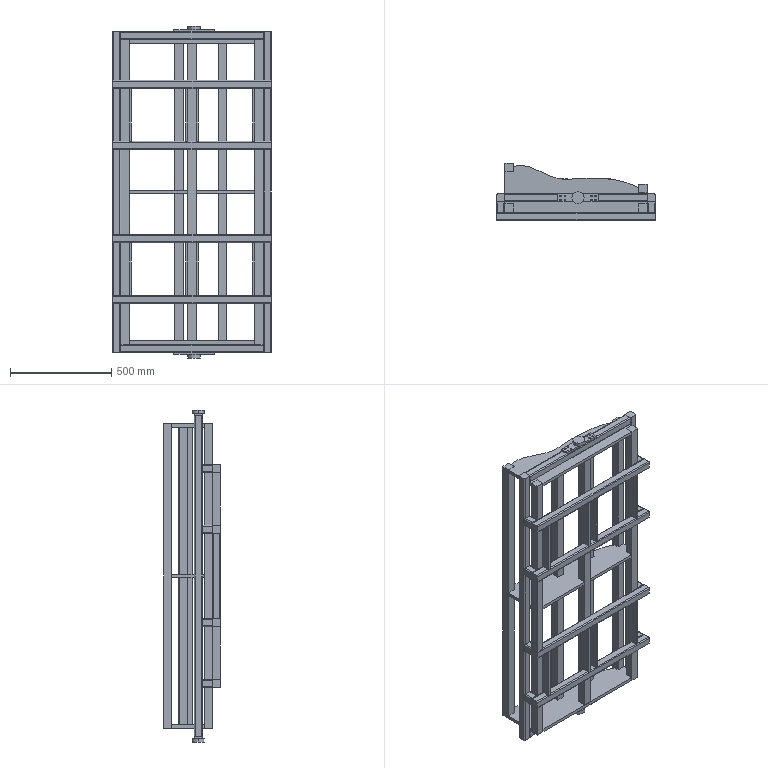Assembly | SolidWorks | mm | 37 component files | 37 solids | 434 faces | box 780 x 280 x 1636 mm | volume 37094171 mm3 | plane 293 | cylinder 104 | cone 32 | spline 5 | commonest cylinder face diameters 10 x68 6.147 x32 60 x4
Bill of materials:
Jig4040-1580 | 2 | Copper | Long, slender straight bar with a square cross-section and rounded longitudinal edges.
Jig4040-420 | 1 | Copper | Straight bar with a square cross-section and rounded longitudinal edges. It is stockier than unnamed part.
Jig4040-50 | 8 | Copper | Short block with a square cross-section and rounded longitudinal edges.
Jig4040-700 | 2 | Copper | Long, straight bar with a square cross-section and rounded longitudinal edges.
Jig4040-780 | 4 | Copper | Long, straight bar with a square cross-section and rounded longitudinal edges.
JigBaffle | 8 | Copper | Flat rectangular strip with both corners chamfered at one end, giving a tapered tip.
MiddlePlate | 1 |  | Thin flat plate with an irregular outline: curved, wavy edges, stepped rectangular tabs at both ends, and several rectangular notches along both long edges.
SidePlate | 2 |  | Thin flat plate with an irregular outline: a smooth wavy upper edge and stepped rectangular tabs at both ends. Unlike unnamed part, it has no notches between the ends.
SupportBar | 3 |  | Long, slender straight bar with a square cross-section and sharp edges.
TieRod | 4 |  | Long, slender straight bar with a square cross-section and sharp edges.
Two-AxisRotation | 2 |  | Flat rectangular plate with a raised cylindrical boss in the middle and eight small round holes, four at each end in a 2x2 pattern. The boss diameter is wider than the plate.
Mates:
1. coincident | Jig4040-1580-1 face at (11.992, -17.909, 2370) dir (1, 0, 0) | Jig4040-700-1 face at (11.992, 17.091, 2365) dir (-1, 0, 0)
2. coincident | Jig4040-1580-1 face at (-28.008, 22.091, 2370) dir (0, 1, 0) | Jig4040-700-1 face at (711.992, 22.091, 2365) dir (0, 1, 0)
3. coincident | Jig4040-1580-1 face at (-28.008, -17.909, 2370) dir (0, 0, 1) | Jig4040-700-1 face at (711.992, -12.909, 2370) dir (0, 0, 1)
4. coincident | Jig4040-1580-1 face at (-28.008, 22.091, 2370) dir (0, 1, 0) | Jig4040-700-2 face at (711.992, 22.091, 825) dir (0, 1, 0)
5. coincident | Jig4040-1580-1 face at (11.992, -17.909, 2370) dir (1, 0, 0) | Jig4040-700-2 face at (11.992, 17.091, 825) dir (-1, 0, 0)
6. coincident | Jig4040-1580-1 face at (-28.008, -17.909, 790) dir (0, 0, -1) | Jig4040-700-2 face at (711.992, -12.909, 790) dir (0, 0, -1)
7. coincident | Jig4040-700-1 face at (711.992, 22.091, 2365) dir (0, 1, 0) | Jig4040-1580-2 face at (711.992, 22.091, 2370) dir (0, 1, 0)
8. coincident | Jig4040-700-1 face at (711.992, -12.909, 2370) dir (0, 0, 1) | Jig4040-1580-2 face at (711.992, -17.909, 2370) dir (0, 0, 1)
9. coincident | Jig4040-700-1 face at (711.992, 17.091, 2365) dir (1, 0, 0) | Jig4040-1580-2 face at (711.992, -17.909, 2370) dir (-1, 0, 0)
10. coincident | Jig4040-700-1 face at (711.992, -12.909, 2330) dir (0, 0, -1) | SofaBackrest-1/SidePlate-2 face at (358.165, 95.613, 2330) dir (0, 0, 1)
11. coincident | Jig4040-1580-2 face at (711.992, -17.909, 2370) dir (-1, 0, 0) | SofaBackrest-1/TieRod-4 face at (711.992, 69.219, 2330) dir (1, 0, 0)
12. distance | SofaBackrest-1/TieRod-3 face at (671.992, -67.909, 2330) dir (0, -1, 0) | Jig4040-1580-2 face at (711.992, -17.909, 2370) dir (0, -1, 0)
13. coincident | Jig4040-1580-1 face at (-28.008, -17.909, 2370) dir (0, -1, 0) | Jig4040-50-1 face at (-23.008, -17.909, 2125) dir (0, 1, 0)
14. coincident | Jig4040-1580-1 face at (-28.008, -17.909, 2370) dir (-1, 0, 0) | Jig4040-50-1 face at (-28.008, -17.909, 2125) dir (-1, 0, 0)
15. coincident | Jig4040-1580-1 face at (-28.008, -17.909, 2370) dir (0, -1, 0) | Jig4040-50-2 face at (-23.008, -17.909, 1065) dir (0, 1, 0)
16. coincident | Jig4040-1580-1 face at (-28.008, -17.909, 2370) dir (-1, 0, 0) | Jig4040-50-2 face at (-28.008, -17.909, 1065) dir (-1, 0, 0)
17. distance | Jig4040-50-2 face at (-23.008, -17.909, 1030) dir (0, 0, -1) | Jig4040-1580-1 face at (-28.008, -17.909, 790) dir (0, 0, -1)
18. distance | Jig4040-50-1 face at (-23.008, -17.909, 2130) dir (0, 0, 1) | Jig4040-1580-1 face at (-28.008, -17.909, 2370) dir (0, 0, 1)
19. coincident | Jig4040-1580-1 face at (-28.008, -17.909, 2370) dir (0, -1, 0) | Jig4040-50-3 face at (-23.008, -17.909, 1365) dir (0, 1, 0)
20. coincident | Jig4040-50-2 face at (-28.008, -17.909, 1065) dir (-1, 0, 0) | Jig4040-50-3 face at (-28.008, -17.909, 1365) dir (-1, 0, 0)
21. coincident | Jig4040-1580-1 face at (-28.008, -17.909, 2370) dir (0, -1, 0) | Jig4040-50-4 face at (-23.008, -17.909, 1825) dir (0, 1, 0)
22. coincident | Jig4040-50-1 face at (-28.008, -17.909, 2125) dir (-1, 0, 0) | Jig4040-50-4 face at (-28.008, -17.909, 1825) dir (-1, 0, 0)
23. distance | Jig4040-50-4 face at (-23.008, -17.909, 1830) dir (0, 0, 1) | Jig4040-50-1 face at (-23.008, -17.909, 2090) dir (0, 0, -1)
24. distance | Jig4040-50-2 face at (-23.008, -17.909, 1070) dir (0, 0, 1) | Jig4040-50-3 face at (-23.008, -17.909, 1330) dir (0, 0, -1)
25. coincident | Jig4040-1580-2 face at (751.992, -17.909, 2370) dir (1, 0, 0) | Jig4040-50-5 face at (751.992, -17.909, 2125) dir (1, 0, 0)
26. coincident | Jig4040-1580-2 face at (711.992, -17.909, 2370) dir (0, -1, 0) | Jig4040-50-5 face at (716.992, -17.909, 2125) dir (0, 1, 0)
27. coincident | Jig4040-50-1 face at (-23.008, -17.909, 2130) dir (0, 0, 1) | Jig4040-50-5 face at (716.992, -17.909, 2130) dir (0, 0, 1)
28. coincident | Jig4040-1580-2 face at (751.992, -17.909, 2370) dir (1, 0, 0) | Jig4040-50-6 face at (751.992, -17.909, 1825) dir (1, 0, 0)
29. coincident | Jig4040-1580-2 face at (751.992, -17.909, 2370) dir (1, 0, 0) | Jig4040-50-7 face at (751.992, -17.909, 1365) dir (1, 0, 0)
30. coincident | Jig4040-1580-2 face at (751.992, -17.909, 2370) dir (1, 0, 0) | Jig4040-50-8 face at (751.992, -17.909, 1065) dir (1, 0, 0)
31. coincident | Jig4040-1580-2 face at (711.992, -17.909, 2370) dir (0, -1, 0) | Jig4040-50-6 face at (716.992, -17.909, 1825) dir (0, 1, 0)
32. coincident | Jig4040-1580-2 face at (711.992, -17.909, 2370) dir (0, -1, 0) | Jig4040-50-7 face at (716.992, -17.909, 1365) dir (0, 1, 0)
33. coincident | Jig4040-1580-2 face at (711.992, -17.909, 2370) dir (0, -1, 0) | Jig4040-50-8 face at (716.992, -17.909, 1065) dir (0, 1, 0)
34. coincident | Jig4040-50-2 face at (-23.008, -17.909, 1070) dir (0, 0, 1) | Jig4040-50-8 face at (716.992, -17.909, 1070) dir (0, 0, 1)
35. coincident | Jig4040-50-3 face at (-23.008, -17.909, 1370) dir (0, 0, 1) | Jig4040-50-7 face at (716.992, -17.909, 1370) dir (0, 0, 1)
36. coincident | Jig4040-50-4 face at (-23.008, -17.909, 1830) dir (0, 0, 1) | Jig4040-50-6 face at (716.992, -17.909, 1830) dir (0, 0, 1)
37. coincident | Jig4040-50-8 face at (716.992, -67.909, 1065) dir (0, -1, 0) | Jig4040-780-1 face at (-28.008, -67.909, 1035) dir (0, 1, 0)
38. coincident | Jig4040-50-8 face at (751.992, -17.909, 1065) dir (1, 0, 0) | Jig4040-780-1 face at (751.992, -102.909, 1035) dir (1, 0, 0)
39. coincident | Jig4040-50-8 face at (716.992, -17.909, 1070) dir (0, 0, 1) | Jig4040-780-1 face at (-28.008, -102.909, 1070) dir (0, 0, 1)
40. coincident | Jig4040-50-3 face at (-23.008, -67.909, 1365) dir (0, -1, 0) | Jig4040-780-2 face at (751.992, -67.909, 1365) dir (0, 1, 0)
41. coincident | Jig4040-50-3 face at (-23.008, -17.909, 1370) dir (0, 0, 1) | Jig4040-780-2 face at (751.992, -102.909, 1370) dir (0, 0, 1)
42. coincident | Jig4040-50-7 face at (751.992, -17.909, 1365) dir (1, 0, 0) | Jig4040-780-2 face at (751.992, -102.909, 1365) dir (1, 0, 0)
43. coincident | Jig4040-50-6 face at (716.992, -67.909, 1825) dir (0, -1, 0) | Jig4040-780-3 face at (751.992, -67.909, 1825) dir (0, 1, 0)
44. coincident | Jig4040-50-4 face at (-23.008, -17.909, 1830) dir (0, 0, 1) | Jig4040-780-3 face at (751.992, -102.909, 1830) dir (0, 0, 1)
45. coincident | Jig4040-50-4 face at (-28.008, -17.909, 1825) dir (-1, 0, 0) | Jig4040-780-3 face at (-28.008, -102.909, 1825) dir (-1, 0, 0)
46. coincident | Jig4040-50-5 face at (716.992, -67.909, 2125) dir (0, -1, 0) | Jig4040-780-4 face at (751.992, -67.909, 2125) dir (0, 1, 0)
47. coincident | Jig4040-50-5 face at (716.992, -17.909, 2090) dir (0, 0, -1) | Jig4040-780-4 face at (751.992, -102.909, 2090) dir (0, 0, -1)
48. coincident | Jig4040-50-5 face at (751.992, -17.909, 2125) dir (1, 0, 0) | Jig4040-780-4 face at (751.992, -102.909, 2125) dir (1, 0, 0)
49. coincident | Jig4040-780-2 face at (751.992, -107.909, 1365) dir (0, -1, 0) | JigBaffle-1 face at (51.992, -107.909, 1330) dir (0, -1, 0)
50. coincident | Jig4040-780-2 face at (751.992, -102.909, 1330) dir (0, 0, -1) | JigBaffle-1 face at (51.992, -107.909, 1330) dir (0, 0, 1)
51. coincident | SofaBackrest-1/TieRod-2 face at (51.992, -27.909, 2330) dir (1, 0, 0) | JigBaffle-1 face at (51.992, -107.909, 1330) dir (-1, 0, 0)
52. coincident | Jig4040-780-1 face at (-28.008, -107.909, 1035) dir (0, -1, 0) | JigBaffle-2 face at (331.992, -107.909, 1330) dir (0, -1, 0)
53. coincident | Jig4040-780-2 face at (751.992, -102.909, 1330) dir (0, 0, -1) | JigBaffle-2 face at (331.992, -107.909, 1330) dir (0, 0, 1)
54. coincident | SofaBackrest-1/SupportBar-2 face at (341.992, -27.909, 2314) dir (-1, 0, 0) | JigBaffle-2 face at (341.992, -107.909, 1330) dir (1, 0, 0)
55. coincident | Jig4040-780-2 face at (751.992, -107.909, 1365) dir (0, -1, 0) | JigBaffle-3 face at (381.992, -107.909, 1330) dir (0, -1, 0)
56. coincident | Jig4040-780-1 face at (-28.008, -102.909, 1070) dir (0, 0, 1) | JigBaffle-3 face at (381.992, -107.909, 1070) dir (0, 0, -1)
57. coincident | SofaBackrest-1/SupportBar-2 face at (381.992, -27.909, 2314) dir (1, 0, 0) | JigBaffle-3 face at (381.992, -107.909, 1330) dir (-1, 0, 0)
58. coincident | Jig4040-780-1 face at (-28.008, -107.909, 1035) dir (0, -1, 0) | JigBaffle-4 face at (661.992, -107.909, 1330) dir (0, -1, 0)
59. coincident | Jig4040-780-1 face at (-28.008, -102.909, 1070) dir (0, 0, 1) | JigBaffle-4 face at (661.992, -107.909, 1070) dir (0, 0, -1)
60. coincident | SofaBackrest-1/TieRod-3 face at (671.992, -27.909, 2330) dir (-1, 0, 0) | JigBaffle-4 face at (671.992, -107.909, 1330) dir (1, 0, 0)
61. coincident | Jig4040-780-4 face at (751.992, -107.909, 2125) dir (0, -1, 0) | JigBaffle-5 face at (51.992, -107.909, 2090) dir (0, -1, 0)
62. coincident | Jig4040-780-3 face at (751.992, -102.909, 1830) dir (0, 0, 1) | JigBaffle-5 face at (51.992, -107.909, 1830) dir (0, 0, -1)
63. coincident | SofaBackrest-1/TieRod-2 face at (51.992, -27.909, 2330) dir (1, 0, 0) | JigBaffle-5 face at (51.992, -107.909, 2090) dir (-1, 0, 0)
64. coincident | Jig4040-700-1 face at (711.992, -12.909, 2370) dir (0, 0, 1) | Two-AxisRotation-1 face at (271.992, -17.909, 2370) dir (0, 0, -1)
65. coincident | Jig4040-700-1 face at (711.992, 22.091, 2365) dir (0, 1, 0) | Two-AxisRotation-1 face at (271.992, 22.091, 2380) dir (0, 1, 0)
66. distance | Two-AxisRotation-1 face at (271.992, -17.909, 2380) dir (-1, 0, 0) | Jig4040-1580-1 face at (-28.008, -17.909, 2370) dir (-1, 0, 0)
67. coincident | Jig4040-700-2 face at (711.992, -12.909, 790) dir (0, 0, -1) | Two-AxisRotation-2 face at (471.992, -17.909, 790) dir (0, 0, 1)
68. coincident | Jig4040-700-2 face at (711.992, 22.091, 825) dir (0, 1, 0) | Two-AxisRotation-2 face at (471.992, 22.091, 780) dir (0, 1, 0)
69. distance | Two-AxisRotation-2 face at (271.992, -17.909, 780) dir (-1, 0, 0) | Jig4040-1580-1 face at (-28.008, -17.909, 2370) dir (-1, 0, 0)
70. coincident | Jig4040-780-4 face at (751.992, -107.909, 2125) dir (0, -1, 0) | JigBaffle-6 face at (381.992, -107.909, 2090) dir (0, -1, 0)
71. coincident | Jig4040-780-4 face at (751.992, -102.909, 2090) dir (0, 0, -1) | JigBaffle-6 face at (381.992, -107.909, 2090) dir (0, 0, 1)
72. coincident | SofaBackrest-1/SupportBar-2 face at (381.992, -27.909, 2314) dir (1, 0, 0) | JigBaffle-6 face at (381.992, -107.909, 2090) dir (-1, 0, 0)
73. coincident | Jig4040-780-4 face at (751.992, -107.909, 2125) dir (0, -1, 0) | JigBaffle-7 face at (331.992, -107.909, 2090) dir (0, -1, 0)
74. coincident | Jig4040-780-3 face at (751.992, -102.909, 1830) dir (0, 0, 1) | JigBaffle-7 face at (331.992, -107.909, 1830) dir (0, 0, -1)
75. coincident | SofaBackrest-1/SupportBar-2 face at (341.992, -27.909, 2314) dir (-1, 0, 0) | JigBaffle-7 face at (341.992, -107.909, 2090) dir (1, 0, 0)
76. coincident | SofaBackrest-1/TieRod-3 face at (671.992, -27.909, 2330) dir (-1, 0, 0) | JigBaffle-8 face at (671.992, -107.909, 2090) dir (1, 0, 0)
77. coincident | Jig4040-780-3 face at (751.992, -102.909, 1830) dir (0, 0, 1) | JigBaffle-8 face at (661.992, -107.909, 1830) dir (0, 0, -1)
78. coincident | Jig4040-780-4 face at (751.992, -107.909, 2125) dir (0, -1, 0) | JigBaffle-8 face at (661.992, -107.909, 2090) dir (0, -1, 0)
79. coincident | Jig4040-780-2 face at (-28.008, -102.909, 1365) dir (-1, 0, 0) | Jig4040-420-1 face at (-28.008, -102.909, 1790) dir (-1, 0, 0)
80. coincident | Jig4040-780-3 face at (751.992, -102.909, 1790) dir (0, 0, -1) | Jig4040-420-1 face at (-23.008, -72.909, 1790) dir (0, 0, 1)
81. coincident | Jig4040-780-2 face at (751.992, -107.909, 1365) dir (0, -1, 0) | Jig4040-420-1 face at (-23.008, -107.909, 1790) dir (0, -1, 0)
82. coincident | SidePlate-1 face at (-71.948, 36.297, -8) dir (0, 0, -1) | TieRod-1 face at (-385.456, 94.081, -8) dir (0, 0, -1)
83. coincident | SidePlate-1 face at (-418.121, -87.225, 8) dir (-1, 0, 0) | TieRod-1 face at (-418.121, 112.775, 1492) dir (-1, 0, 0)
84. coincident | SidePlate-1 face at (-418.121, 72.775, 8) dir (0, 1, 0) | TieRod-1 face at (-418.121, 72.775, 1492) dir (0, -1, 0)
85. coincident | SidePlate-1 face at (-418.121, -87.225, 8) dir (0, -1, 0) | TieRod-2 face at (-418.121, -87.225, 1492) dir (0, 1, 0)
86. coincident | SidePlate-1 face at (-418.121, -87.225, 8) dir (-1, 0, 0) | TieRod-2 face at (-418.121, -87.225, 1492) dir (-1, 0, 0)
87. coincident | SidePlate-1 face at (-71.948, 36.297, -8) dir (0, 0, -1) | TieRod-2 face at (-385.456, -105.919, -8) dir (0, 0, -1)
88. coincident | SidePlate-1 face at (281.879, -30.097, 8) dir (1, 0, 0) | TieRod-4 face at (281.879, 9.903, 1492) dir (1, 0, 0)
89. coincident | SidePlate-1 face at (-71.948, 36.297, -8) dir (0, 0, -1) | TieRod-4 face at (274.544, -8.79, -8) dir (0, 0, -1)
90. coincident | SidePlate-1 face at (281.879, -30.097, 8) dir (1, 0, 0) | TieRod-3 face at (281.879, -87.225, 1492) dir (1, 0, 0)
91. coincident | SidePlate-1 face at (-71.948, 36.297, -8) dir (0, 0, -1) | TieRod-3 face at (274.544, -105.919, -8) dir (0, 0, -1)
92. coincident | SidePlate-1 face at (-378.121, -127.225, 8) dir (0, -1, 0) | TieRod-3 face at (241.879, -127.225, 1492) dir (0, -1, 0)
93. coincident | SidePlate-1 face at (281.879, -30.097, 8) dir (0, 1, 0) | TieRod-4 face at (241.879, -30.097, 1492) dir (0, -1, 0)
94. coincident | TieRod-1 face at (-385.456, 94.081, 1492) dir (0, 0, 1) | SidePlate-2 face at (-71.948, 36.297, 1492) dir (0, 0, 1)
95. coincident | TieRod-2 face at (-418.121, -127.225, 1492) dir (0, -1, 0) | SidePlate-2 face at (-378.121, -127.225, 1492) dir (0, -1, 0)
96. coincident | TieRod-2 face at (-418.121, -87.225, 1492) dir (-1, 0, 0) | SidePlate-2 face at (-418.121, -87.225, 1492) dir (-1, 0, 0)
97. coincident | TieRod-2 face at (-418.121, -87.225, 1492) dir (-1, 0, 0) | MiddlePlate-1 face at (-418.121, -87.225, 750) dir (-1, 0, 0)
98. coincident | TieRod-2 face at (-418.121, -127.225, 1492) dir (0, -1, 0) | MiddlePlate-1 face at (-378.121, -127.225, 750) dir (0, -1, 0)
99. distance | MiddlePlate-1 face at (-264.174, 82.239, 750) dir (0, 0, 1) | SidePlate-2 face at (-71.948, 36.297, 1476) dir (0, 0, -1)
100. coincident | SupportBar-1 face at (-119.629, 17.592, 1476) dir (0, 0, 1) | SupportBar-2 face at (-55.456, -105.919, 1476) dir (0, 0, 1)
101. coincident | SupportBar-2 face at (-55.456, -105.919, 1476) dir (0, 0, 1) | SupportBar-3 face at (94.51, 20.069, 1476) dir (0, 0, 1)
102. coincident | SidePlate-2 face at (-71.948, 36.297, 1476) dir (0, 0, -1) | SupportBar-2 face at (-55.456, -105.919, 1476) dir (0, 0, 1)
103. coincident | MiddlePlate-1 face at (-152.294, 36.782, 750) dir (1, 0, 0) | SupportBar-1 face at (-152.294, 36.286, 1476) dir (-1, 0, 0)
104. coincident | MiddlePlate-1 face at (-88.121, -127.225, 750) dir (1, 0, 0) | SupportBar-2 face at (-88.121, -87.225, 1476) dir (-1, 0, 0)
105. coincident | MiddlePlate-1 face at (61.845, 38.84, 750) dir (1, 0, 0) | SupportBar-3 face at (61.845, 38.763, 1476) dir (-1, 0, 0)
106. coincident | MiddlePlate-1 face at (-378.121, -127.225, 750) dir (0, -1, 0) | SupportBar-2 face at (-88.121, -127.225, 1476) dir (0, -1, 0)
107. coincident | MiddlePlate-1 edge at (-152.294, -3.714, 750) dir (0, 0, -1) | SupportBar-1 edge at (-152.294, -3.714, 1476) dir (0, 0, -1)
108. coincident | MiddlePlate-1 edge at (61.845, -1.237, 750) dir (0, 0, -1) | SupportBar-3 edge at (61.845, -1.237, 1476) dir (0, 0, -1)